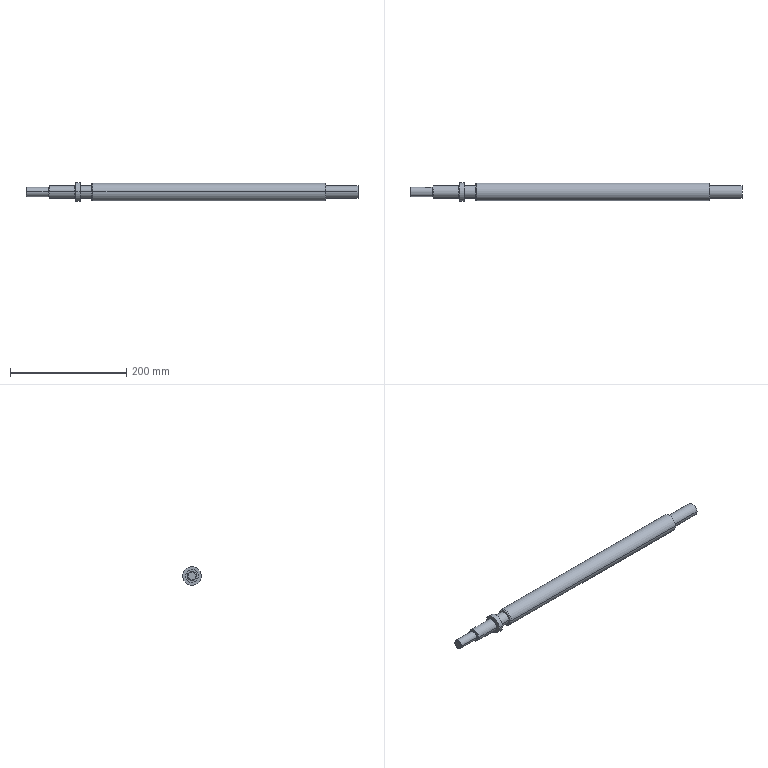Component | SolidWorks | 3LeadScrew-1 | 1 solid | 37 faces | box 570 x 32 x 32 mm | volume 343727 mm3 | cylinder 19 | plane 12 | cone 6 | commonest cylinder face diameters 22 x6 5 x3 16 x2 15 x2 21 x2 32 x2 30 x2
STEP:
#1=COLOUR_RGB('',0.7922,0.8196,0.9333);
#2=FILL_AREA_STYLE_COLOUR('',#1);
#3=FILL_AREA_STYLE('',(#2));
#4=SURFACE_STYLE_FILL_AREA(#3);
#5=SURFACE_SIDE_STYLE('',(#4));
#6=SURFACE_STYLE_USAGE(.BOTH.,#5);
#7=PRESENTATION_STYLE_ASSIGNMENT((#6));
#8=CARTESIAN_POINT('',(-12.116,2.748,-0.005406));
#9=VERTEX_POINT('',#8);
#10=CARTESIAN_POINT('',(-12.214,2.745,-0.1038));
#11=VERTEX_POINT('',#10);
#12=CARTESIAN_POINT('',(-12.214,2.748,-0.005406));
#13=DIRECTION('',(-0.,0.9996,-0.02861));
#14=DIRECTION('',(1.,0.,0.));
#15=AXIS2_PLACEMENT_3D('',#12,#13,#14);
#16=CIRCLE('',#15,0.09843);
#17=EDGE_CURVE('',#9,#11,#16,.T.);
#18=ORIENTED_EDGE('',*,*,#17,.F.);
#19=CARTESIAN_POINT('',(-12.116,2.874,-0.00901));
#20=VERTEX_POINT('',#19);
#21=CARTESIAN_POINT('',(-12.116,2.748,-0.005406));
#22=DIRECTION('',(-0.,0.9996,-0.02861));
#23=VECTOR('',#22,39.37);
#24=LINE('',#21,#23);
#25=EDGE_CURVE('',#9,#20,#24,.T.);
#26=ORIENTED_EDGE('',*,*,#25,.T.);
#27=CARTESIAN_POINT('',(-12.214,2.855,-0.1069));
#28=VERTEX_POINT('',#27);
#29=CARTESIAN_POINT('',(-12.214,2.855,-0.1069));
#30=CARTESIAN_POINT('',(-12.208,2.855,-0.1069));
#31=CARTESIAN_POINT('',(-12.201,2.856,-0.1063));
#32=CARTESIAN_POINT('',(-12.189,2.856,-0.1038));
#33=CARTESIAN_POINT('',(-12.182,2.857,-0.1019));
#34=CARTESIAN_POINT('',(-12.171,2.859,-0.09699));
#35=CARTESIAN_POINT('',(-12.165,2.86,-0.09399));
#36=CARTESIAN_POINT('',(-12.154,2.862,-0.0869));
#37=CARTESIAN_POINT('',(-12.149,2.863,-0.08281));
#38=CARTESIAN_POINT('',(-12.136,2.866,-0.06937));
#39=CARTESIAN_POINT('',(-12.128,2.869,-0.05851));
#40=CARTESIAN_POINT('',(-12.121,2.871,-0.04082));
#41=CARTESIAN_POINT('',(-12.119,2.872,-0.03459));
#42=CARTESIAN_POINT('',(-12.117,2.873,-0.02189));
#43=CARTESIAN_POINT('',(-12.116,2.874,-0.01548));
#44=CARTESIAN_POINT('',(-12.116,2.874,-0.00901));
#45=B_SPLINE_CURVE_WITH_KNOTS('',3,(#29,#30,#31,#32,#33,#34,#35,#36,#37,#38,#39,#40,#41,#42,#43,#44),.UNSPECIFIED.,.F.,.F.,(4,2,2,2,2,2,2,4),(0.,0.0004917,0.0009835,0.001475,0.001967,0.00295,0.003442,0.003934),.UNSPECIFIED.);
#46=EDGE_CURVE('',#28,#20,#45,.T.);
#47=ORIENTED_EDGE('',*,*,#46,.F.);
#48=CARTESIAN_POINT('',(-12.214,2.745,-0.1038));
#49=DIRECTION('',(-0.,0.9996,-0.02861));
#50=VECTOR('',#49,39.37);
#51=LINE('',#48,#50);
#52=EDGE_CURVE('',#11,#28,#51,.T.);
#53=ORIENTED_EDGE('',*,*,#52,.F.);
#54=EDGE_LOOP('',(#18,#26,#47,#53));
#55=FACE_OUTER_BOUND('',#54,.T.);
#56=CARTESIAN_POINT('',(-12.214,2.748,-0.005406));
#57=DIRECTION('',(-0.,0.9996,-0.02861));
#58=DIRECTION('',(1.,0.,0.));
#59=AXIS2_PLACEMENT_3D('',#56,#57,#58);
#60=CYLINDRICAL_SURFACE('',#59,0.09843);
#61=ADVANCED_FACE('',(#55),#60,.F.);
#62=CARTESIAN_POINT('',(-13.583,2.287,0.007791));
#63=VERTEX_POINT('',#62);
#64=CARTESIAN_POINT('',(-13.583,2.831,-0.007791));
#65=VERTEX_POINT('',#64);
#66=CARTESIAN_POINT('',(-13.583,2.559,-0.));
#67=DIRECTION('',(1.,0.,0.));
#68=DIRECTION('',(0.,-0.9996,0.02861));
#69=AXIS2_PLACEMENT_3D('',#66,#67,#68);
#70=CIRCLE('',#69,0.2723);
#71=EDGE_CURVE('',#63,#65,#70,.T.);
#72=ORIENTED_EDGE('',*,*,#71,.T.);
#73=CARTESIAN_POINT('',(-13.54,2.874,-0.00901));
#74=VERTEX_POINT('',#73);
#75=CARTESIAN_POINT('',(-13.583,2.831,-0.007791));
#76=DIRECTION('',(0.7071,0.7068,-0.02023));
#77=VECTOR('',#76,39.37);
#78=LINE('',#75,#77);
#79=EDGE_CURVE('',#65,#74,#78,.T.);
#80=ORIENTED_EDGE('',*,*,#79,.T.);
#81=CARTESIAN_POINT('',(-13.54,2.244,0.00901));
#82=VERTEX_POINT('',#81);
#83=CARTESIAN_POINT('',(-13.54,2.559,-0.));
#84=DIRECTION('',(1.,0.,0.));
#85=DIRECTION('',(0.,-0.9996,0.02861));
#86=AXIS2_PLACEMENT_3D('',#83,#84,#85);
#87=CIRCLE('',#86,0.315);
#88=EDGE_CURVE('',#82,#74,#87,.T.);
#89=ORIENTED_EDGE('',*,*,#88,.F.);
#90=CARTESIAN_POINT('',(-13.583,2.287,0.007791));
#91=DIRECTION('',(0.7071,-0.7068,0.02023));
#92=VECTOR('',#91,39.37);
#93=LINE('',#90,#92);
#94=EDGE_CURVE('',#63,#82,#93,.T.);
#95=ORIENTED_EDGE('',*,*,#94,.F.);
#96=EDGE_LOOP('',(#72,#80,#89,#95));
#97=FACE_OUTER_BOUND('',#96,.T.);
#98=CARTESIAN_POINT('',(-13.583,2.559,-0.));
#99=DIRECTION('',(1.,0.,0.));
#100=DIRECTION('',(0.,-0.9996,0.02861));
#101=AXIS2_PLACEMENT_3D('',#98,#99,#100);
#102=CONICAL_SURFACE('',#101,0.2723,0.7854);
#103=ADVANCED_FACE('',(#97),#102,.T.);
#104=CARTESIAN_POINT('',(-9.134,3.104,-0.01559));
#105=VERTEX_POINT('',#104);
#106=CARTESIAN_POINT('',(-9.134,2.014,0.01559));
#107=VERTEX_POINT('',#106);
#108=CARTESIAN_POINT('',(-9.134,2.559,-0.));
#109=DIRECTION('',(-1.,-0.,-0.));
#110=DIRECTION('',(0.,0.9996,-0.02861));
#111=AXIS2_PLACEMENT_3D('',#108,#109,#110);
#112=CIRCLE('',#111,0.5451);
#113=EDGE_CURVE('',#105,#107,#112,.T.);
#114=ORIENTED_EDGE('',*,*,#113,.F.);
#115=CARTESIAN_POINT('',(-9.055,3.149,-0.01689));
#116=VERTEX_POINT('',#115);
#117=CARTESIAN_POINT('',(-9.134,3.104,-0.01559));
#118=DIRECTION('',(0.866,0.4998,-0.0143));
#119=VECTOR('',#118,39.37);
#120=LINE('',#117,#119);
#121=EDGE_CURVE('',#105,#116,#120,.T.);
#122=ORIENTED_EDGE('',*,*,#121,.T.);
#123=CARTESIAN_POINT('',(-9.055,1.969,0.01689));
#124=VERTEX_POINT('',#123);
#125=CARTESIAN_POINT('',(-9.055,2.559,-0.));
#126=DIRECTION('',(1.,0.,0.));
#127=DIRECTION('',(0.,0.9996,-0.02861));
#128=AXIS2_PLACEMENT_3D('',#125,#126,#127);
#129=CIRCLE('',#128,0.5906);
#130=EDGE_CURVE('',#124,#116,#129,.T.);
#131=ORIENTED_EDGE('',*,*,#130,.F.);
#132=CARTESIAN_POINT('',(-9.134,2.014,0.01559));
#133=DIRECTION('',(0.866,-0.4998,0.0143));
#134=VECTOR('',#133,39.37);
#135=LINE('',#132,#134);
#136=EDGE_CURVE('',#107,#124,#135,.T.);
#137=ORIENTED_EDGE('',*,*,#136,.F.);
#138=EDGE_LOOP('',(#114,#122,#131,#137));
#139=FACE_OUTER_BOUND('',#138,.T.);
#140=CARTESIAN_POINT('',(-9.134,2.559,-0.));
#141=DIRECTION('',(1.,0.,0.));
#142=DIRECTION('',(0.,-0.9996,0.02861));
#143=AXIS2_PLACEMENT_3D('',#140,#141,#142);
#144=CONICAL_SURFACE('',#143,0.5451,0.5236);
#145=ADVANCED_FACE('',(#139),#144,.T.);
#146=CARTESIAN_POINT('',(6.693,2.047,0.01464));
#147=VERTEX_POINT('',#146);
#148=CARTESIAN_POINT('',(6.693,3.071,-0.01464));
#149=VERTEX_POINT('',#148);
#150=CARTESIAN_POINT('',(6.693,2.559,-0.));
#151=DIRECTION('',(1.,0.,0.));
#152=DIRECTION('',(0.,0.9996,-0.02861));
#153=AXIS2_PLACEMENT_3D('',#150,#151,#152);
#154=CIRCLE('',#153,0.5118);
#155=EDGE_CURVE('',#147,#149,#154,.T.);
#156=ORIENTED_EDGE('',*,*,#155,.F.);
#157=CARTESIAN_POINT('',(6.647,1.969,0.01689));
#158=VERTEX_POINT('',#157);
#159=CARTESIAN_POINT('',(6.647,1.969,0.01689));
#160=DIRECTION('',(-0.5,-0.8657,0.02477));
#161=VECTOR('',#160,39.37);
#162=LINE('',#159,#161);
#163=EDGE_CURVE('',#147,#158,#162,.T.);
#164=ORIENTED_EDGE('',*,*,#163,.T.);
#165=CARTESIAN_POINT('',(6.647,3.149,-0.01689));
#166=VERTEX_POINT('',#165);
#167=CARTESIAN_POINT('',(6.647,2.559,-0.));
#168=DIRECTION('',(-1.,-0.,-0.));
#169=DIRECTION('',(0.,0.9996,-0.02861));
#170=AXIS2_PLACEMENT_3D('',#167,#168,#169);
#171=CIRCLE('',#170,0.5906);
#172=EDGE_CURVE('',#166,#158,#171,.T.);
#173=ORIENTED_EDGE('',*,*,#172,.F.);
#174=CARTESIAN_POINT('',(6.647,3.149,-0.01689));
#175=DIRECTION('',(-0.5,0.8657,-0.02477));
#176=VECTOR('',#175,39.37);
#177=LINE('',#174,#176);
#178=EDGE_CURVE('',#149,#166,#177,.T.);
#179=ORIENTED_EDGE('',*,*,#178,.F.);
#180=EDGE_LOOP('',(#156,#164,#173,#179));
#181=FACE_OUTER_BOUND('',#180,.T.);
#182=CARTESIAN_POINT('',(6.647,2.559,-0.));
#183=DIRECTION('',(-1.,-0.,-0.));
#184=DIRECTION('',(0.,0.9996,-0.02861));
#185=AXIS2_PLACEMENT_3D('',#182,#183,#184);
#186=CONICAL_SURFACE('',#185,0.5906,1.047);
#187=ADVANCED_FACE('',(#181),#186,.T.);
#188=ORIENTED_EDGE('',*,*,#88,.T.);
#189=CARTESIAN_POINT('',(-12.588,2.874,-0.00901));
#190=VERTEX_POINT('',#189);
#191=CARTESIAN_POINT('',(-13.583,2.874,-0.00901));
#192=DIRECTION('',(1.,0.,0.));
#193=VECTOR('',#192,39.37);
#194=LINE('',#191,#193);
#195=EDGE_CURVE('',#74,#190,#194,.T.);
#196=ORIENTED_EDGE('',*,*,#195,.T.);
#197=CARTESIAN_POINT('',(-12.49,2.855,-0.1069));
#198=VERTEX_POINT('',#197);
#199=CARTESIAN_POINT('',(-12.588,2.874,-0.00901));
#200=CARTESIAN_POINT('',(-12.588,2.874,-0.01547));
#201=CARTESIAN_POINT('',(-12.588,2.873,-0.02202));
#202=CARTESIAN_POINT('',(-12.585,2.872,-0.03464));
#203=CARTESIAN_POINT('',(-12.583,2.871,-0.04077));
#204=CARTESIAN_POINT('',(-12.578,2.87,-0.05269));
#205=CARTESIAN_POINT('',(-12.575,2.869,-0.05835));
#206=CARTESIAN_POINT('',(-12.568,2.866,-0.0689));
#207=CARTESIAN_POINT('',(-12.564,2.865,-0.07387));
#208=CARTESIAN_POINT('',(-12.555,2.863,-0.08287));
#209=CARTESIAN_POINT('',(-12.55,2.862,-0.08688));
#210=CARTESIAN_POINT('',(-12.539,2.86,-0.09395));
#211=CARTESIAN_POINT('',(-12.534,2.859,-0.09701));
#212=CARTESIAN_POINT('',(-12.522,2.857,-0.1019));
#213=CARTESIAN_POINT('',(-12.516,2.856,-0.1038));
#214=CARTESIAN_POINT('',(-12.503,2.856,-0.1063));
#215=CARTESIAN_POINT('',(-12.496,2.855,-0.1069));
#216=CARTESIAN_POINT('',(-12.49,2.855,-0.1069));
#217=B_SPLINE_CURVE_WITH_KNOTS('',3,(#199,#200,#201,#202,#203,#204,#205,#206,#207,#208,#209,#210,#211,#212,#213,#214,#215,#216),.UNSPECIFIED.,.F.,.F.,(4,2,2,2,2,2,2,2,4),(0.003934,0.004425,0.004916,0.005407,0.005898,0.006389,0.006881,0.007372,0.007863),.UNSPECIFIED.);
#218=EDGE_CURVE('',#190,#198,#217,.T.);
#219=ORIENTED_EDGE('',*,*,#218,.T.);
#220=CARTESIAN_POINT('',(-13.583,2.855,-0.1069));
#221=DIRECTION('',(1.,0.,0.));
#222=VECTOR('',#221,39.37);
#223=LINE('',#220,#222);
#224=EDGE_CURVE('',#198,#28,#223,.T.);
#225=ORIENTED_EDGE('',*,*,#224,.T.);
#226=ORIENTED_EDGE('',*,*,#46,.T.);
#227=CARTESIAN_POINT('',(-12.087,2.874,-0.00901));
#228=VERTEX_POINT('',#227);
#229=CARTESIAN_POINT('',(-13.583,2.874,-0.00901));
#230=DIRECTION('',(1.,0.,0.));
#231=VECTOR('',#230,39.37);
#232=LINE('',#229,#231);
#233=EDGE_CURVE('',#20,#228,#232,.T.);
#234=ORIENTED_EDGE('',*,*,#233,.T.);
#235=CARTESIAN_POINT('',(-12.087,2.244,0.00901));
#236=VERTEX_POINT('',#235);
#237=CARTESIAN_POINT('',(-12.087,2.559,-0.));
#238=DIRECTION('',(-1.,-0.,-0.));
#239=DIRECTION('',(0.,0.9996,-0.02861));
#240=AXIS2_PLACEMENT_3D('',#237,#238,#239);
#241=CIRCLE('',#240,0.315);
#242=EDGE_CURVE('',#228,#236,#241,.T.);
#243=ORIENTED_EDGE('',*,*,#242,.T.);
#244=CARTESIAN_POINT('',(-13.583,2.244,0.00901));
#245=DIRECTION('',(1.,0.,0.));
#246=VECTOR('',#245,39.37);
#247=LINE('',#244,#246);
#248=EDGE_CURVE('',#82,#236,#247,.T.);
#249=ORIENTED_EDGE('',*,*,#248,.F.);
#250=EDGE_LOOP('',(#188,#196,#219,#225,#226,#234,#243,#249));
#251=FACE_OUTER_BOUND('',#250,.T.);
#252=CARTESIAN_POINT('',(-13.583,2.559,-0.));
#253=DIRECTION('',(1.,0.,0.));
#254=DIRECTION('',(0.,-0.9996,0.02861));
#255=AXIS2_PLACEMENT_3D('',#252,#253,#254);
#256=CYLINDRICAL_SURFACE('',#255,0.315);
#257=ADVANCED_FACE('',(#251),#256,.T.);
#258=CARTESIAN_POINT('',(-12.087,2.854,-0.008447));
#259=VERTEX_POINT('',#258);
#260=CARTESIAN_POINT('',(-12.087,2.264,0.008447));
#261=VERTEX_POINT('',#260);
#262=CARTESIAN_POINT('',(-12.087,2.559,-0.));
#263=DIRECTION('',(-1.,-0.,-0.));
#264=DIRECTION('',(0.,0.9996,-0.02861));
#265=AXIS2_PLACEMENT_3D('',#262,#263,#264);
#266=CIRCLE('',#265,0.2953);
#267=EDGE_CURVE('',#259,#261,#266,.T.);
#268=ORIENTED_EDGE('',*,*,#267,.F.);
#269=CARTESIAN_POINT('',(-12.008,2.854,-0.008447));
#270=VERTEX_POINT('',#269);
#271=CARTESIAN_POINT('',(-12.087,2.854,-0.008447));
#272=DIRECTION('',(1.,0.,0.));
#273=VECTOR('',#272,39.37);
#274=LINE('',#271,#273);
#275=EDGE_CURVE('',#259,#270,#274,.T.);
#276=ORIENTED_EDGE('',*,*,#275,.T.);
#277=CARTESIAN_POINT('',(-12.008,2.264,0.008447));
#278=VERTEX_POINT('',#277);
#279=CARTESIAN_POINT('',(-12.008,2.559,-0.));
#280=DIRECTION('',(-1.,-0.,-0.));
#281=DIRECTION('',(0.,0.9996,-0.02861));
#282=AXIS2_PLACEMENT_3D('',#279,#280,#281);
#283=CIRCLE('',#282,0.2953);
#284=EDGE_CURVE('',#270,#278,#283,.T.);
#285=ORIENTED_EDGE('',*,*,#284,.T.);
#286=CARTESIAN_POINT('',(-12.087,2.264,0.008447));
#287=DIRECTION('',(1.,0.,0.));
#288=VECTOR('',#287,39.37);
#289=LINE('',#286,#288);
#290=EDGE_CURVE('',#261,#278,#289,.T.);
#291=ORIENTED_EDGE('',*,*,#290,.F.);
#292=EDGE_LOOP('',(#268,#276,#285,#291));
#293=FACE_OUTER_BOUND('',#292,.T.);
#294=CARTESIAN_POINT('',(-12.087,2.559,-0.));
#295=DIRECTION('',(1.,0.,0.));
#296=DIRECTION('',(0.,-0.9996,0.02861));
#297=AXIS2_PLACEMENT_3D('',#294,#295,#296);
#298=CYLINDRICAL_SURFACE('',#297,0.2953);
#299=ADVANCED_FACE('',(#293),#298,.T.);
#300=CARTESIAN_POINT('',(-12.008,2.992,-0.01239));
#301=VERTEX_POINT('',#300);
#302=CARTESIAN_POINT('',(-12.008,2.126,0.01239));
#303=VERTEX_POINT('',#302);
#304=CARTESIAN_POINT('',(-12.008,2.559,-0.));
#305=DIRECTION('',(-1.,-0.,-0.));
#306=DIRECTION('',(0.,0.9996,-0.02861));
#307=AXIS2_PLACEMENT_3D('',#304,#305,#306);
#308=CIRCLE('',#307,0.4331);
#309=EDGE_CURVE('',#301,#303,#308,.T.);
#310=ORIENTED_EDGE('',*,*,#309,.F.);
#311=CARTESIAN_POINT('',(-10.315,2.992,-0.01239));
#312=VERTEX_POINT('',#311);
#313=CARTESIAN_POINT('',(-12.008,2.992,-0.01239));
#314=DIRECTION('',(1.,0.,0.));
#315=VECTOR('',#314,39.37);
#316=LINE('',#313,#315);
#317=EDGE_CURVE('',#301,#312,#316,.T.);
#318=ORIENTED_EDGE('',*,*,#317,.T.);
#319=CARTESIAN_POINT('',(-10.315,2.126,0.01239));
#320=VERTEX_POINT('',#319);
#321=CARTESIAN_POINT('',(-10.315,2.559,-0.));
#322=DIRECTION('',(-1.,-0.,-0.));
#323=DIRECTION('',(0.,0.9996,-0.02861));
#324=AXIS2_PLACEMENT_3D('',#321,#322,#323);
#325=CIRCLE('',#324,0.4331);
#326=EDGE_CURVE('',#312,#320,#325,.T.);
#327=ORIENTED_EDGE('',*,*,#326,.T.);
#328=CARTESIAN_POINT('',(-12.008,2.126,0.01239));
#329=DIRECTION('',(1.,0.,0.));
#330=VECTOR('',#329,39.37);
#331=LINE('',#328,#330);
#332=EDGE_CURVE('',#303,#320,#331,.T.);
#333=ORIENTED_EDGE('',*,*,#332,.F.);
#334=EDGE_LOOP('',(#310,#318,#327,#333));
#335=FACE_OUTER_BOUND('',#334,.T.);
#336=CARTESIAN_POINT('',(-12.008,2.559,-0.));
#337=DIRECTION('',(1.,0.,0.));
#338=DIRECTION('',(0.,-0.9996,0.02861));
#339=AXIS2_PLACEMENT_3D('',#336,#337,#338);
#340=CYLINDRICAL_SURFACE('',#339,0.4331);
#341=ADVANCED_FACE('',(#335),#340,.T.);
#342=CARTESIAN_POINT('',(-10.315,2.972,-0.01183));
#343=VERTEX_POINT('',#342);
#344=CARTESIAN_POINT('',(-10.315,2.146,0.01183));
#345=VERTEX_POINT('',#344);
#346=CARTESIAN_POINT('',(-10.315,2.559,-0.));
#347=DIRECTION('',(-1.,-0.,-0.));
#348=DIRECTION('',(0.,0.9996,-0.02861));
#349=AXIS2_PLACEMENT_3D('',#346,#347,#348);
#350=CIRCLE('',#349,0.4134);
#351=EDGE_CURVE('',#343,#345,#350,.T.);
#352=ORIENTED_EDGE('',*,*,#351,.F.);
#353=CARTESIAN_POINT('',(-10.236,2.972,-0.01183));
#354=VERTEX_POINT('',#353);
#355=CARTESIAN_POINT('',(-10.315,2.972,-0.01183));
#356=DIRECTION('',(1.,0.,0.));
#357=VECTOR('',#356,39.37);
#358=LINE('',#355,#357);
#359=EDGE_CURVE('',#343,#354,#358,.T.);
#360=ORIENTED_EDGE('',*,*,#359,.T.);
#361=CARTESIAN_POINT('',(-10.236,2.146,0.01183));
#362=VERTEX_POINT('',#361);
#363=CARTESIAN_POINT('',(-10.236,2.559,-0.));
#364=DIRECTION('',(-1.,-0.,-0.));
#365=DIRECTION('',(0.,0.9996,-0.02861));
#366=AXIS2_PLACEMENT_3D('',#363,#364,#365);
#367=CIRCLE('',#366,0.4134);
#368=EDGE_CURVE('',#354,#362,#367,.T.);
#369=ORIENTED_EDGE('',*,*,#368,.T.);
#370=CARTESIAN_POINT('',(-10.315,2.146,0.01183));
#371=DIRECTION('',(1.,0.,0.));
#372=VECTOR('',#371,39.37);
#373=LINE('',#370,#372);
#374=EDGE_CURVE('',#345,#362,#373,.T.);
#375=ORIENTED_EDGE('',*,*,#374,.F.);
#376=EDGE_LOOP('',(#352,#360,#369,#375));
#377=FACE_OUTER_BOUND('',#376,.T.);
#378=CARTESIAN_POINT('',(-10.315,2.559,-0.));
#379=DIRECTION('',(1.,0.,0.));
#380=DIRECTION('',(0.,-0.9996,0.02861));
#381=AXIS2_PLACEMENT_3D('',#378,#379,#380);
#382=CYLINDRICAL_SURFACE('',#381,0.4134);
#383=ADVANCED_FACE('',(#377),#382,.T.);
#384=CARTESIAN_POINT('',(-10.236,3.189,-0.01802));
#385=VERTEX_POINT('',#384);
#386=CARTESIAN_POINT('',(-10.236,1.929,0.01802));
#387=VERTEX_POINT('',#386);
#388=CARTESIAN_POINT('',(-10.236,2.559,-0.));
#389=DIRECTION('',(-1.,-0.,-0.));
#390=DIRECTION('',(0.,0.9996,-0.02861));
#391=AXIS2_PLACEMENT_3D('',#388,#389,#390);
#392=CIRCLE('',#391,0.6299);
#393=EDGE_CURVE('',#385,#387,#392,.T.);
#394=ORIENTED_EDGE('',*,*,#393,.F.);
#395=CARTESIAN_POINT('',(-9.921,3.189,-0.01802));
#396=VERTEX_POINT('',#395);
#397=CARTESIAN_POINT('',(-10.236,3.189,-0.01802));
#398=DIRECTION('',(1.,0.,0.));
#399=VECTOR('',#398,39.37);
#400=LINE('',#397,#399);
#401=EDGE_CURVE('',#385,#396,#400,.T.);
#402=ORIENTED_EDGE('',*,*,#401,.T.);
#403=CARTESIAN_POINT('',(-9.921,1.929,0.01802));
#404=VERTEX_POINT('',#403);
#405=CARTESIAN_POINT('',(-9.921,2.559,-0.));
#406=DIRECTION('',(-1.,-0.,-0.));
#407=DIRECTION('',(0.,0.9996,-0.02861));
#408=AXIS2_PLACEMENT_3D('',#405,#406,#407);
#409=CIRCLE('',#408,0.6299);
#410=EDGE_CURVE('',#396,#404,#409,.T.);
#411=ORIENTED_EDGE('',*,*,#410,.T.);
#412=CARTESIAN_POINT('',(-10.236,1.929,0.01802));
#413=DIRECTION('',(1.,0.,0.));
#414=VECTOR('',#413,39.37);
#415=LINE('',#412,#414);
#416=EDGE_CURVE('',#387,#404,#415,.T.);
#417=ORIENTED_EDGE('',*,*,#416,.F.);
#418=EDGE_LOOP('',(#394,#402,#411,#417));
#419=FACE_OUTER_BOUND('',#418,.T.);
#420=CARTESIAN_POINT('',(-10.236,2.559,-0.));
#421=DIRECTION('',(1.,0.,0.));
#422=DIRECTION('',(0.,-0.9996,0.02861));
#423=AXIS2_PLACEMENT_3D('',#420,#421,#422);
#424=CYLINDRICAL_SURFACE('',#423,0.6299);
#425=ADVANCED_FACE('',(#419),#424,.T.);
#426=CARTESIAN_POINT('',(-9.921,2.992,-0.01239));
#427=VERTEX_POINT('',#426);
#428=CARTESIAN_POINT('',(-9.921,2.126,0.01239));
#429=VERTEX_POINT('',#428);
#430=CARTESIAN_POINT('',(-9.921,2.559,-0.));
#431=DIRECTION('',(-1.,-0.,-0.));
#432=DIRECTION('',(0.,0.9996,-0.02861));
#433=AXIS2_PLACEMENT_3D('',#430,#431,#432);
#434=CIRCLE('',#433,0.4331);
#435=EDGE_CURVE('',#427,#429,#434,.T.);
#436=ORIENTED_EDGE('',*,*,#435,.F.);
#437=CARTESIAN_POINT('',(-9.134,2.992,-0.01239));
#438=VERTEX_POINT('',#437);
#439=CARTESIAN_POINT('',(-9.921,2.992,-0.01239));
#440=DIRECTION('',(1.,0.,0.));
#441=VECTOR('',#440,39.37);
#442=LINE('',#439,#441);
#443=EDGE_CURVE('',#427,#438,#442,.T.);
#444=ORIENTED_EDGE('',*,*,#443,.T.);
#445=CARTESIAN_POINT('',(-9.134,2.126,0.01239));
#446=VERTEX_POINT('',#445);
#447=CARTESIAN_POINT('',(-9.134,2.559,-0.));
#448=DIRECTION('',(-1.,-0.,-0.));
#449=DIRECTION('',(0.,0.9996,-0.02861));
#450=AXIS2_PLACEMENT_3D('',#447,#448,#449);
#451=CIRCLE('',#450,0.4331);
#452=EDGE_CURVE('',#438,#446,#451,.T.);
#453=ORIENTED_EDGE('',*,*,#452,.T.);
#454=CARTESIAN_POINT('',(-9.921,2.126,0.01239));
#455=DIRECTION('',(1.,0.,0.));
#456=VECTOR('',#455,39.37);
#457=LINE('',#454,#456);
#458=EDGE_CURVE('',#429,#446,#457,.T.);
#459=ORIENTED_EDGE('',*,*,#458,.F.);
#460=EDGE_LOOP('',(#436,#444,#453,#459));
#461=FACE_OUTER_BOUND('',#460,.T.);
#462=CARTESIAN_POINT('',(-9.921,2.559,-0.));
#463=DIRECTION('',(1.,0.,0.));
#464=DIRECTION('',(0.,-0.9996,0.02861));
#465=AXIS2_PLACEMENT_3D('',#462,#463,#464);
#466=CYLINDRICAL_SURFACE('',#465,0.4331);
#467=ADVANCED_FACE('',(#461),#466,.T.);
#468=ORIENTED_EDGE('',*,*,#130,.T.);
#469=CARTESIAN_POINT('',(-9.134,3.149,-0.01689));
#470=DIRECTION('',(1.,0.,0.));
#471=VECTOR('',#470,39.37);
#472=LINE('',#469,#471);
#473=EDGE_CURVE('',#116,#166,#472,.T.);
#474=ORIENTED_EDGE('',*,*,#473,.T.);
#475=ORIENTED_EDGE('',*,*,#172,.T.);
#476=CARTESIAN_POINT('',(-9.134,1.969,0.01689));
#477=DIRECTION('',(1.,0.,0.));
#478=VECTOR('',#477,39.37);
#479=LINE('',#476,#478);
#480=EDGE_CURVE('',#124,#158,#479,.T.);
#481=ORIENTED_EDGE('',*,*,#480,.F.);
#482=EDGE_LOOP('',(#468,#474,#475,#481));
#483=FACE_OUTER_BOUND('',#482,.T.);
#484=CARTESIAN_POINT('',(-9.134,2.559,-0.));
#485=DIRECTION('',(1.,0.,0.));
#486=DIRECTION('',(0.,-0.9996,0.02861));
#487=AXIS2_PLACEMENT_3D('',#484,#485,#486);
#488=CYLINDRICAL_SURFACE('',#487,0.5906);
#489=ADVANCED_FACE('',(#483),#488,.T.);
#490=CARTESIAN_POINT('',(6.693,2.992,-0.01239));
#491=VERTEX_POINT('',#490);
#492=CARTESIAN_POINT('',(6.693,2.126,0.01239));
#493=VERTEX_POINT('',#492);
#494=CARTESIAN_POINT('',(6.693,2.559,-0.));
#495=DIRECTION('',(-1.,-0.,-0.));
#496=DIRECTION('',(0.,0.9996,-0.02861));
#497=AXIS2_PLACEMENT_3D('',#494,#495,#496);
#498=CIRCLE('',#497,0.4331);
#499=EDGE_CURVE('',#491,#493,#498,.T.);
#500=ORIENTED_EDGE('',*,*,#499,.F.);
#501=CARTESIAN_POINT('',(8.858,2.992,-0.01239));
#502=VERTEX_POINT('',#501);
#503=CARTESIAN_POINT('',(6.693,2.992,-0.01239));
#504=DIRECTION('',(1.,0.,0.));
#505=VECTOR('',#504,39.37);
#506=LINE('',#503,#505);
#507=EDGE_CURVE('',#491,#502,#506,.T.);
#508=ORIENTED_EDGE('',*,*,#507,.T.);
#509=CARTESIAN_POINT('',(8.858,2.126,0.01239));
#510=VERTEX_POINT('',#509);
#511=CARTESIAN_POINT('',(8.858,2.559,-0.));
#512=DIRECTION('',(-1.,-0.,-0.));
#513=DIRECTION('',(0.,0.9996,-0.02861));
#514=AXIS2_PLACEMENT_3D('',#511,#512,#513);
#515=CIRCLE('',#514,0.4331);
#516=EDGE_CURVE('',#502,#510,#515,.T.);
#517=ORIENTED_EDGE('',*,*,#516,.T.);
#518=CARTESIAN_POINT('',(6.693,2.126,0.01239));
#519=DIRECTION('',(1.,0.,0.));
#520=VECTOR('',#519,39.37);
#521=LINE('',#518,#520);
#522=EDGE_CURVE('',#493,#510,#521,.T.);
#523=ORIENTED_EDGE('',*,*,#522,.F.);
#524=EDGE_LOOP('',(#500,#508,#517,#523));
#525=FACE_OUTER_BOUND('',#524,.T.);
#526=CARTESIAN_POINT('',(6.693,2.559,-0.));
#527=DIRECTION('',(1.,0.,0.));
#528=DIRECTION('',(0.,-0.9996,0.02861));
#529=AXIS2_PLACEMENT_3D('',#526,#527,#528);
#530=CYLINDRICAL_SURFACE('',#529,0.4331);
#531=ADVANCED_FACE('',(#525),#530,.T.);
#532=ORIENTED_EDGE('',*,*,#507,.F.);
#533=CARTESIAN_POINT('',(6.693,2.559,-0.));
#534=DIRECTION('',(-1.,-0.,-0.));
#535=DIRECTION('',(0.,0.9996,-0.02861));
#536=AXIS2_PLACEMENT_3D('',#533,#534,#535);
#537=CIRCLE('',#536,0.4331);
#538=EDGE_CURVE('',#493,#491,#537,.T.);
#539=ORIENTED_EDGE('',*,*,#538,.F.);
#540=ORIENTED_EDGE('',*,*,#522,.T.);
#541=CARTESIAN_POINT('',(8.858,2.559,-0.));
#542=DIRECTION('',(-1.,-0.,-0.));
#543=DIRECTION('',(0.,0.9996,-0.02861));
#544=AXIS2_PLACEMENT_3D('',#541,#542,#543);
#545=CIRCLE('',#544,0.4331);
#546=EDGE_CURVE('',#510,#502,#545,.T.);
#547=ORIENTED_EDGE('',*,*,#546,.T.);
#548=EDGE_LOOP('',(#532,#539,#540,#547));
#549=FACE_OUTER_BOUND('',#548,.T.);
#550=CARTESIAN_POINT('',(6.693,2.559,-0.));
#551=DIRECTION('',(1.,0.,0.));
#552=DIRECTION('',(0.,-0.9996,0.02861));
#553=AXIS2_PLACEMENT_3D('',#550,#551,#552);
#554=CYLINDRICAL_SURFACE('',#553,0.4331);
#555=ADVANCED_FACE('',(#549),#554,.T.);
#556=ORIENTED_EDGE('',*,*,#546,.F.);
#557=ORIENTED_EDGE('',*,*,#516,.F.);
#558=EDGE_LOOP('',(#556,#557));
#559=FACE_OUTER_BOUND('',#558,.T.);
#560=CARTESIAN_POINT('',(8.858,2.559,-0.));
#561=DIRECTION('',(-1.,-0.,-0.));
#562=DIRECTION('',(-0.,0.9996,-0.02861));
#563=AXIS2_PLACEMENT_3D('',#560,#561,#562);
#564=PLANE('',#563);
#565=ADVANCED_FACE('',(#559),#564,.F.);
#566=ORIENTED_EDGE('',*,*,#473,.F.);
#567=CARTESIAN_POINT('',(-9.055,2.559,-0.));
#568=DIRECTION('',(1.,0.,0.));
#569=DIRECTION('',(0.,0.9996,-0.02861));
#570=AXIS2_PLACEMENT_3D('',#567,#568,#569);
#571=CIRCLE('',#570,0.5906);
#572=EDGE_CURVE('',#116,#124,#571,.T.);
#573=ORIENTED_EDGE('',*,*,#572,.T.);
#574=ORIENTED_EDGE('',*,*,#480,.T.);
#575=CARTESIAN_POINT('',(6.647,2.559,-0.));
#576=DIRECTION('',(-1.,-0.,-0.));
#577=DIRECTION('',(0.,0.9996,-0.02861));
#578=AXIS2_PLACEMENT_3D('',#575,#576,#577);
#579=CIRCLE('',#578,0.5906);
#580=EDGE_CURVE('',#158,#166,#579,.T.);
#581=ORIENTED_EDGE('',*,*,#580,.T.);
#582=EDGE_LOOP('',(#566,#573,#574,#581));
#583=FACE_OUTER_BOUND('',#582,.T.);
#584=CARTESIAN_POINT('',(-9.134,2.559,-0.));
#585=DIRECTION('',(1.,0.,0.));
#586=DIRECTION('',(0.,-0.9996,0.02861));
#587=AXIS2_PLACEMENT_3D('',#584,#585,#586);
#588=CYLINDRICAL_SURFACE('',#587,0.5906);
#589=ADVANCED_FACE('',(#583),#588,.T.);
#590=CARTESIAN_POINT('',(-9.134,2.559,-0.));
#591=DIRECTION('',(-1.,-0.,-0.));
#592=DIRECTION('',(0.,0.9996,-0.02861));
#593=AXIS2_PLACEMENT_3D('',#590,#591,#592);
#594=CIRCLE('',#593,0.5451);
#595=EDGE_CURVE('',#107,#105,#594,.T.);
#596=ORIENTED_EDGE('',*,*,#595,.T.);
#597=ORIENTED_EDGE('',*,*,#113,.T.);
#598=EDGE_LOOP('',(#596,#597));
#599=FACE_OUTER_BOUND('',#598,.T.);
#600=CARTESIAN_POINT('',(-9.134,2.559,-0.));
#601=DIRECTION('',(-1.,-0.,-0.));
#602=DIRECTION('',(0.,0.9996,-0.02861));
#603=AXIS2_PLACEMENT_3D('',#600,#601,#602);
#604=CIRCLE('',#603,0.4331);
#605=EDGE_CURVE('',#446,#438,#604,.T.);
#606=ORIENTED_EDGE('',*,*,#605,.F.);
#607=ORIENTED_EDGE('',*,*,#452,.F.);
#608=EDGE_LOOP('',(#606,#607));
#609=FACE_BOUND('',#608,.T.);
#610=CARTESIAN_POINT('',(-9.134,2.559,-0.));
#611=DIRECTION('',(-1.,-0.,-0.));
#612=DIRECTION('',(-0.,0.9996,-0.02861));
#613=AXIS2_PLACEMENT_3D('',#610,#611,#612);
#614=PLANE('',#613);
#615=ADVANCED_FACE('',(#599,#609),#614,.T.);
#616=CARTESIAN_POINT('',(6.693,2.559,-0.));
#617=DIRECTION('',(1.,0.,0.));
#618=DIRECTION('',(0.,0.9996,-0.02861));
#619=AXIS2_PLACEMENT_3D('',#616,#617,#618);
#620=CIRCLE('',#619,0.5118);
#621=EDGE_CURVE('',#149,#147,#620,.T.);
#622=ORIENTED_EDGE('',*,*,#621,.T.);
#623=ORIENTED_EDGE('',*,*,#155,.T.);
#624=EDGE_LOOP('',(#622,#623));
#625=FACE_OUTER_BOUND('',#624,.T.);
#626=ORIENTED_EDGE('',*,*,#538,.T.);
#627=ORIENTED_EDGE('',*,*,#499,.T.);
#628=EDGE_LOOP('',(#626,#627));
#629=FACE_BOUND('',#628,.T.);
#630=CARTESIAN_POINT('',(6.693,2.559,-0.));
#631=DIRECTION('',(-1.,-0.,-0.));
#632=DIRECTION('',(-0.,0.9996,-0.02861));
#633=AXIS2_PLACEMENT_3D('',#630,#631,#632);
#634=PLANE('',#633);
#635=ADVANCED_FACE('',(#625,#629),#634,.F.);
#636=ORIENTED_EDGE('',*,*,#443,.F.);
#637=CARTESIAN_POINT('',(-9.921,2.559,-0.));
#638=DIRECTION('',(-1.,-0.,-0.));
#639=DIRECTION('',(0.,0.9996,-0.02861));
#640=AXIS2_PLACEMENT_3D('',#637,#638,#639);
#641=CIRCLE('',#640,0.4331);
#642=EDGE_CURVE('',#429,#427,#641,.T.);
#643=ORIENTED_EDGE('',*,*,#642,.F.);
#644=ORIENTED_EDGE('',*,*,#458,.T.);
#645=ORIENTED_EDGE('',*,*,#605,.T.);
#646=EDGE_LOOP('',(#636,#643,#644,#645));
#647=FACE_OUTER_BOUND('',#646,.T.);
#648=CARTESIAN_POINT('',(-9.921,2.559,-0.));
#649=DIRECTION('',(1.,0.,0.));
#650=DIRECTION('',(0.,-0.9996,0.02861));
#651=AXIS2_PLACEMENT_3D('',#648,#649,#650);
#652=CYLINDRICAL_SURFACE('',#651,0.4331);
#653=ADVANCED_FACE('',(#647),#652,.T.);
#654=ORIENTED_EDGE('',*,*,#401,.F.);
#655=CARTESIAN_POINT('',(-10.236,2.559,-0.));
#656=DIRECTION('',(-1.,-0.,-0.));
#657=DIRECTION('',(0.,0.9996,-0.02861));
#658=AXIS2_PLACEMENT_3D('',#655,#656,#657);
#659=CIRCLE('',#658,0.6299);
#660=EDGE_CURVE('',#387,#385,#659,.T.);
#661=ORIENTED_EDGE('',*,*,#660,.F.);
#662=ORIENTED_EDGE('',*,*,#416,.T.);
#663=CARTESIAN_POINT('',(-9.921,2.559,-0.));
#664=DIRECTION('',(-1.,-0.,-0.));
#665=DIRECTION('',(0.,0.9996,-0.02861));
#666=AXIS2_PLACEMENT_3D('',#663,#664,#665);
#667=CIRCLE('',#666,0.6299);
#668=EDGE_CURVE('',#404,#396,#667,.T.);
#669=ORIENTED_EDGE('',*,*,#668,.T.);
#670=EDGE_LOOP('',(#654,#661,#662,#669));
#671=FACE_OUTER_BOUND('',#670,.T.);
#672=CARTESIAN_POINT('',(-10.236,2.559,-0.));
#673=DIRECTION('',(1.,0.,0.));
#674=DIRECTION('',(0.,-0.9996,0.02861));
#675=AXIS2_PLACEMENT_3D('',#672,#673,#674);
#676=CYLINDRICAL_SURFACE('',#675,0.6299);
#677=ADVANCED_FACE('',(#671),#676,.T.);
#678=CARTESIAN_POINT('',(-10.236,2.559,-0.));
#679=DIRECTION('',(-1.,-0.,-0.));
#680=DIRECTION('',(0.,0.9996,-0.02861));
#681=AXIS2_PLACEMENT_3D('',#678,#679,#680);
#682=CIRCLE('',#681,0.4134);
#683=EDGE_CURVE('',#362,#354,#682,.T.);
#684=ORIENTED_EDGE('',*,*,#683,.F.);
#685=ORIENTED_EDGE('',*,*,#368,.F.);
#686=EDGE_LOOP('',(#684,#685));
#687=FACE_BOUND('',#686,.T.);
#688=ORIENTED_EDGE('',*,*,#660,.T.);
#689=ORIENTED_EDGE('',*,*,#393,.T.);
#690=EDGE_LOOP('',(#688,#689));
#691=FACE_OUTER_BOUND('',#690,.T.);
#692=CARTESIAN_POINT('',(-10.236,2.559,-0.));
#693=DIRECTION('',(-1.,-0.,-0.));
#694=DIRECTION('',(-0.,0.9996,-0.02861));
#695=AXIS2_PLACEMENT_3D('',#692,#693,#694);
#696=PLANE('',#695);
#697=ADVANCED_FACE('',(#687,#691),#696,.T.);
#698=ORIENTED_EDGE('',*,*,#642,.T.);
#699=ORIENTED_EDGE('',*,*,#435,.T.);
#700=EDGE_LOOP('',(#698,#699));
#701=FACE_BOUND('',#700,.T.);
#702=ORIENTED_EDGE('',*,*,#668,.F.);
#703=ORIENTED_EDGE('',*,*,#410,.F.);
#704=EDGE_LOOP('',(#702,#703));
#705=FACE_OUTER_BOUND('',#704,.T.);
#706=CARTESIAN_POINT('',(-9.921,2.559,-0.));
#707=DIRECTION('',(-1.,-0.,-0.));
#708=DIRECTION('',(-0.,0.9996,-0.02861));
#709=AXIS2_PLACEMENT_3D('',#706,#707,#708);
#710=PLANE('',#709);
#711=ADVANCED_FACE('',(#701,#705),#710,.F.);
#712=ORIENTED_EDGE('',*,*,#359,.F.);
#713=CARTESIAN_POINT('',(-10.315,2.559,-0.));
#714=DIRECTION('',(-1.,-0.,-0.));
#715=DIRECTION('',(0.,0.9996,-0.02861));
#716=AXIS2_PLACEMENT_3D('',#713,#714,#715);
#717=CIRCLE('',#716,0.4134);
#718=EDGE_CURVE('',#345,#343,#717,.T.);
#719=ORIENTED_EDGE('',*,*,#718,.F.);
#720=ORIENTED_EDGE('',*,*,#374,.T.);
#721=ORIENTED_EDGE('',*,*,#683,.T.);
#722=EDGE_LOOP('',(#712,#719,#720,#721));
#723=FACE_OUTER_BOUND('',#722,.T.);
#724=CARTESIAN_POINT('',(-10.315,2.559,-0.));
#725=DIRECTION('',(1.,0.,0.));
#726=DIRECTION('',(0.,-0.9996,0.02861));
#727=AXIS2_PLACEMENT_3D('',#724,#725,#726);
#728=CYLINDRICAL_SURFACE('',#727,0.4134);
#729=ADVANCED_FACE('',(#723),#728,.T.);
#730=ORIENTED_EDGE('',*,*,#317,.F.);
#731=CARTESIAN_POINT('',(-12.008,2.559,-0.));
#732=DIRECTION('',(-1.,-0.,-0.));
#733=DIRECTION('',(0.,0.9996,-0.02861));
#734=AXIS2_PLACEMENT_3D('',#731,#732,#733);
#735=CIRCLE('',#734,0.4331);
#736=EDGE_CURVE('',#303,#301,#735,.T.);
#737=ORIENTED_EDGE('',*,*,#736,.F.);
#738=ORIENTED_EDGE('',*,*,#332,.T.);
#739=CARTESIAN_POINT('',(-10.315,2.559,-0.));
#740=DIRECTION('',(-1.,-0.,-0.));
#741=DIRECTION('',(0.,0.9996,-0.02861));
#742=AXIS2_PLACEMENT_3D('',#739,#740,#741);
#743=CIRCLE('',#742,0.4331);
#744=EDGE_CURVE('',#320,#312,#743,.T.);
#745=ORIENTED_EDGE('',*,*,#744,.T.);
#746=EDGE_LOOP('',(#730,#737,#738,#745));
#747=FACE_OUTER_BOUND('',#746,.T.);
#748=CARTESIAN_POINT('',(-12.008,2.559,-0.));
#749=DIRECTION('',(1.,0.,0.));
#750=DIRECTION('',(0.,-0.9996,0.02861));
#751=AXIS2_PLACEMENT_3D('',#748,#749,#750);
#752=CYLINDRICAL_SURFACE('',#751,0.4331);
#753=ADVANCED_FACE('',(#747),#752,.T.);
#754=CARTESIAN_POINT('',(-12.008,2.559,-0.));
#755=DIRECTION('',(-1.,-0.,-0.));
#756=DIRECTION('',(0.,0.9996,-0.02861));
#757=AXIS2_PLACEMENT_3D('',#754,#755,#756);
#758=CIRCLE('',#757,0.2953);
#759=EDGE_CURVE('',#278,#270,#758,.T.);
#760=ORIENTED_EDGE('',*,*,#759,.F.);
#761=ORIENTED_EDGE('',*,*,#284,.F.);
#762=EDGE_LOOP('',(#760,#761));
#763=FACE_BOUND('',#762,.T.);
#764=ORIENTED_EDGE('',*,*,#736,.T.);
#765=ORIENTED_EDGE('',*,*,#309,.T.);
#766=EDGE_LOOP('',(#764,#765));
#767=FACE_OUTER_BOUND('',#766,.T.);
#768=CARTESIAN_POINT('',(-12.008,2.559,-0.));
#769=DIRECTION('',(-1.,-0.,-0.));
#770=DIRECTION('',(-0.,0.9996,-0.02861));
#771=AXIS2_PLACEMENT_3D('',#768,#769,#770);
#772=PLANE('',#771);
#773=ADVANCED_FACE('',(#763,#767),#772,.T.);
#774=ORIENTED_EDGE('',*,*,#718,.T.);
#775=ORIENTED_EDGE('',*,*,#351,.T.);
#776=EDGE_LOOP('',(#774,#775));
#777=FACE_BOUND('',#776,.T.);
#778=ORIENTED_EDGE('',*,*,#744,.F.);
#779=ORIENTED_EDGE('',*,*,#326,.F.);
#780=EDGE_LOOP('',(#778,#779));
#781=FACE_OUTER_BOUND('',#780,.T.);
#782=CARTESIAN_POINT('',(-10.315,2.559,-0.));
#783=DIRECTION('',(-1.,-0.,-0.));
#784=DIRECTION('',(-0.,0.9996,-0.02861));
#785=AXIS2_PLACEMENT_3D('',#782,#783,#784);
#786=PLANE('',#785);
#787=ADVANCED_FACE('',(#777,#781),#786,.F.);
#788=ORIENTED_EDGE('',*,*,#275,.F.);
#789=CARTESIAN_POINT('',(-12.087,2.559,-0.));
#790=DIRECTION('',(-1.,-0.,-0.));
#791=DIRECTION('',(0.,0.9996,-0.02861));
#792=AXIS2_PLACEMENT_3D('',#789,#790,#791);
#793=CIRCLE('',#792,0.2953);
#794=EDGE_CURVE('',#261,#259,#793,.T.);
#795=ORIENTED_EDGE('',*,*,#794,.F.);
#796=ORIENTED_EDGE('',*,*,#290,.T.);
#797=ORIENTED_EDGE('',*,*,#759,.T.);
#798=EDGE_LOOP('',(#788,#795,#796,#797));
#799=FACE_OUTER_BOUND('',#798,.T.);
#800=CARTESIAN_POINT('',(-12.087,2.559,-0.));
#801=DIRECTION('',(1.,0.,0.));
#802=DIRECTION('',(0.,-0.9996,0.02861));
#803=AXIS2_PLACEMENT_3D('',#800,#801,#802);
#804=CYLINDRICAL_SURFACE('',#803,0.2953);
#805=ADVANCED_FACE('',(#799),#804,.T.);
#806=ORIENTED_EDGE('',*,*,#195,.F.);
#807=CARTESIAN_POINT('',(-13.54,2.559,-0.));
#808=DIRECTION('',(1.,0.,0.));
#809=DIRECTION('',(0.,-0.9996,0.02861));
#810=AXIS2_PLACEMENT_3D('',#807,#808,#809);
#811=CIRCLE('',#810,0.315);
#812=EDGE_CURVE('',#74,#82,#811,.T.);
#813=ORIENTED_EDGE('',*,*,#812,.T.);
#814=ORIENTED_EDGE('',*,*,#248,.T.);
#815=CARTESIAN_POINT('',(-12.087,2.559,-0.));
#816=DIRECTION('',(-1.,-0.,-0.));
#817=DIRECTION('',(0.,0.9996,-0.02861));
#818=AXIS2_PLACEMENT_3D('',#815,#816,#817);
#819=CIRCLE('',#818,0.315);
#820=EDGE_CURVE('',#236,#228,#819,.T.);
#821=ORIENTED_EDGE('',*,*,#820,.T.);
#822=ORIENTED_EDGE('',*,*,#233,.F.);
#823=CARTESIAN_POINT('',(-12.214,2.861,0.08983));
#824=VERTEX_POINT('',#823);
#825=CARTESIAN_POINT('',(-12.116,2.874,-0.00901));
#826=CARTESIAN_POINT('',(-12.116,2.874,-0.002552));
#827=CARTESIAN_POINT('',(-12.117,2.874,0.004013));
#828=CARTESIAN_POINT('',(-12.119,2.874,0.01668));
#829=CARTESIAN_POINT('',(-12.121,2.873,0.02284));
#830=CARTESIAN_POINT('',(-12.126,2.872,0.03484));
#831=CARTESIAN_POINT('',(-12.129,2.871,0.04055));
#832=CARTESIAN_POINT('',(-12.136,2.87,0.05121));
#833=CARTESIAN_POINT('',(-12.14,2.869,0.05624));
#834=CARTESIAN_POINT('',(-12.149,2.867,0.06536));
#835=CARTESIAN_POINT('',(-12.154,2.866,0.06943));
#836=CARTESIAN_POINT('',(-12.165,2.865,0.0766));
#837=CARTESIAN_POINT('',(-12.171,2.864,0.07971));
#838=CARTESIAN_POINT('',(-12.182,2.862,0.08468));
#839=CARTESIAN_POINT('',(-12.189,2.862,0.08658));
#840=CARTESIAN_POINT('',(-12.201,2.861,0.08916));
#841=CARTESIAN_POINT('',(-12.208,2.861,0.08983));
#842=CARTESIAN_POINT('',(-12.214,2.861,0.08983));
#843=B_SPLINE_CURVE_WITH_KNOTS('',3,(#825,#826,#827,#828,#829,#830,#831,#832,#833,#834,#835,#836,#837,#838,#839,#840,#841,#842),.UNSPECIFIED.,.F.,.F.,(4,2,2,2,2,2,2,2,4),(0.003934,0.004425,0.004916,0.005407,0.005898,0.006389,0.006881,0.007372,0.007863),.UNSPECIFIED.);
#844=EDGE_CURVE('',#20,#824,#843,.T.);
#845=ORIENTED_EDGE('',*,*,#844,.T.);
#846=CARTESIAN_POINT('',(-12.49,2.861,0.08983));
#847=VERTEX_POINT('',#846);
#848=CARTESIAN_POINT('',(-13.583,2.861,0.08983));
#849=DIRECTION('',(-1.,-0.,-0.));
#850=VECTOR('',#849,39.37);
#851=LINE('',#848,#850);
#852=EDGE_CURVE('',#824,#847,#851,.T.);
#853=ORIENTED_EDGE('',*,*,#852,.T.);
#854=CARTESIAN_POINT('',(-12.49,2.861,0.08983));
#855=CARTESIAN_POINT('',(-12.496,2.861,0.08983));
#856=CARTESIAN_POINT('',(-12.503,2.861,0.08917));
#857=CARTESIAN_POINT('',(-12.516,2.862,0.08662));
#858=CARTESIAN_POINT('',(-12.522,2.862,0.08469));
#859=CARTESIAN_POINT('',(-12.534,2.864,0.0797));
#860=CARTESIAN_POINT('',(-12.539,2.865,0.07664));
#861=CARTESIAN_POINT('',(-12.55,2.866,0.06945));
#862=CARTESIAN_POINT('',(-12.555,2.867,0.06529));
#863=CARTESIAN_POINT('',(-12.569,2.87,0.05167));
#864=CARTESIAN_POINT('',(-12.576,2.872,0.0407));
#865=CARTESIAN_POINT('',(-12.583,2.873,0.02289));
#866=CARTESIAN_POINT('',(-12.585,2.874,0.01662));
#867=CARTESIAN_POINT('',(-12.588,2.874,0.003877));
#868=CARTESIAN_POINT('',(-12.588,2.874,-0.002544));
#869=CARTESIAN_POINT('',(-12.588,2.874,-0.00901));
#870=B_SPLINE_CURVE_WITH_KNOTS('',3,(#854,#855,#856,#857,#858,#859,#860,#861,#862,#863,#864,#865,#866,#867,#868,#869),.UNSPECIFIED.,.F.,.F.,(4,2,2,2,2,2,2,4),(0.,0.0004917,0.0009835,0.001475,0.001967,0.00295,0.003442,0.003934),.UNSPECIFIED.);
#871=EDGE_CURVE('',#847,#190,#870,.T.);
#872=ORIENTED_EDGE('',*,*,#871,.T.);
#873=EDGE_LOOP('',(#806,#813,#814,#821,#822,#845,#853,#872));
#874=FACE_OUTER_BOUND('',#873,.T.);
#875=CARTESIAN_POINT('',(-13.583,2.559,-0.));
#876=DIRECTION('',(1.,0.,0.));
#877=DIRECTION('',(0.,-0.9996,0.02861));
#878=AXIS2_PLACEMENT_3D('',#875,#876,#877);
#879=CYLINDRICAL_SURFACE('',#878,0.315);
#880=ADVANCED_FACE('',(#874),#879,.T.);
#881=ORIENTED_EDGE('',*,*,#794,.T.);
#882=ORIENTED_EDGE('',*,*,#267,.T.);
#883=EDGE_LOOP('',(#881,#882));
#884=FACE_BOUND('',#883,.T.);
#885=ORIENTED_EDGE('',*,*,#820,.F.);
#886=ORIENTED_EDGE('',*,*,#242,.F.);
#887=EDGE_LOOP('',(#885,#886));
#888=FACE_OUTER_BOUND('',#887,.T.);
#889=CARTESIAN_POINT('',(-12.087,2.559,-0.));
#890=DIRECTION('',(-1.,-0.,-0.));
#891=DIRECTION('',(-0.,0.9996,-0.02861));
#892=AXIS2_PLACEMENT_3D('',#889,#890,#891);
#893=PLANE('',#892);
#894=ADVANCED_FACE('',(#884,#888),#893,.F.);
#895=ORIENTED_EDGE('',*,*,#163,.F.);
#896=ORIENTED_EDGE('',*,*,#621,.F.);
#897=ORIENTED_EDGE('',*,*,#178,.T.);
#898=ORIENTED_EDGE('',*,*,#580,.F.);
#899=EDGE_LOOP('',(#895,#896,#897,#898));
#900=FACE_OUTER_BOUND('',#899,.T.);
#901=CARTESIAN_POINT('',(6.647,2.559,-0.));
#902=DIRECTION('',(-1.,-0.,-0.));
#903=DIRECTION('',(0.,0.9996,-0.02861));
#904=AXIS2_PLACEMENT_3D('',#901,#902,#903);
#905=CONICAL_SURFACE('',#904,0.5906,1.047);
#906=ADVANCED_FACE('',(#900),#905,.T.);
#907=ORIENTED_EDGE('',*,*,#121,.F.);
#908=ORIENTED_EDGE('',*,*,#595,.F.);
#909=ORIENTED_EDGE('',*,*,#136,.T.);
#910=ORIENTED_EDGE('',*,*,#572,.F.);
#911=EDGE_LOOP('',(#907,#908,#909,#910));
#912=FACE_OUTER_BOUND('',#911,.T.);
#913=CARTESIAN_POINT('',(-9.134,2.559,-0.));
#914=DIRECTION('',(1.,0.,0.));
#915=DIRECTION('',(0.,-0.9996,0.02861));
#916=AXIS2_PLACEMENT_3D('',#913,#914,#915);
#917=CONICAL_SURFACE('',#916,0.5451,0.5236);
#918=ADVANCED_FACE('',(#912),#917,.T.);
#919=ORIENTED_EDGE('',*,*,#79,.F.);
#920=CARTESIAN_POINT('',(-13.583,2.559,-0.));
#921=DIRECTION('',(1.,0.,0.));
#922=DIRECTION('',(0.,-0.9996,0.02861));
#923=AXIS2_PLACEMENT_3D('',#920,#921,#922);
#924=CIRCLE('',#923,0.2723);
#925=EDGE_CURVE('',#65,#63,#924,.T.);
#926=ORIENTED_EDGE('',*,*,#925,.T.);
#927=ORIENTED_EDGE('',*,*,#94,.T.);
#928=ORIENTED_EDGE('',*,*,#812,.F.);
#929=EDGE_LOOP('',(#919,#926,#927,#928));
#930=FACE_OUTER_BOUND('',#929,.T.);
#931=CARTESIAN_POINT('',(-13.583,2.559,-0.));
#932=DIRECTION('',(1.,0.,0.));
#933=DIRECTION('',(0.,-0.9996,0.02861));
#934=AXIS2_PLACEMENT_3D('',#931,#932,#933);
#935=CONICAL_SURFACE('',#934,0.2723,0.7854);
#936=ADVANCED_FACE('',(#930),#935,.T.);
#937=ORIENTED_EDGE('',*,*,#71,.F.);
#938=ORIENTED_EDGE('',*,*,#925,.F.);
#939=EDGE_LOOP('',(#937,#938));
#940=FACE_OUTER_BOUND('',#939,.T.);
#941=CARTESIAN_POINT('',(-13.583,2.559,-0.));
#942=DIRECTION('',(-1.,-0.,-0.));
#943=DIRECTION('',(-0.,0.9996,-0.02861));
#944=AXIS2_PLACEMENT_3D('',#941,#942,#943);
#945=PLANE('',#944);
#946=ADVANCED_FACE('',(#940),#945,.T.);
#947=CARTESIAN_POINT('',(-12.49,2.751,0.09298));
#948=VERTEX_POINT('',#947);
#949=CARTESIAN_POINT('',(-12.49,2.751,0.09298));
#950=DIRECTION('',(-0.,0.9996,-0.02861));
#951=VECTOR('',#950,39.37);
#952=LINE('',#949,#951);
#953=EDGE_CURVE('',#948,#847,#952,.T.);
#954=ORIENTED_EDGE('',*,*,#953,.F.);
#955=CARTESIAN_POINT('',(-12.49,2.745,-0.1038));
#956=VERTEX_POINT('',#955);
#957=CARTESIAN_POINT('',(-12.49,2.748,-0.005406));
#958=DIRECTION('',(-0.,0.9996,-0.02861));
#959=DIRECTION('',(1.,0.,0.));
#960=AXIS2_PLACEMENT_3D('',#957,#958,#959);
#961=CIRCLE('',#960,0.09843);
#962=EDGE_CURVE('',#956,#948,#961,.T.);
#963=ORIENTED_EDGE('',*,*,#962,.F.);
#964=CARTESIAN_POINT('',(-12.49,2.745,-0.1038));
#965=DIRECTION('',(-0.,0.9996,-0.02861));
#966=VECTOR('',#965,39.37);
#967=LINE('',#964,#966);
#968=EDGE_CURVE('',#956,#198,#967,.T.);
#969=ORIENTED_EDGE('',*,*,#968,.T.);
#970=ORIENTED_EDGE('',*,*,#218,.F.);
#971=ORIENTED_EDGE('',*,*,#871,.F.);
#972=EDGE_LOOP('',(#954,#963,#969,#970,#971));
#973=FACE_OUTER_BOUND('',#972,.T.);
#974=CARTESIAN_POINT('',(-12.49,2.748,-0.005406));
#975=DIRECTION('',(-0.,0.9996,-0.02861));
#976=DIRECTION('',(1.,0.,0.));
#977=AXIS2_PLACEMENT_3D('',#974,#975,#976);
#978=CYLINDRICAL_SURFACE('',#977,0.09843);
#979=ADVANCED_FACE('',(#973),#978,.F.);
#980=ORIENTED_EDGE('',*,*,#968,.F.);
#981=CARTESIAN_POINT('',(-12.49,2.745,-0.1038));
#982=DIRECTION('',(-1.,-0.,-0.));
#983=VECTOR('',#982,39.37);
#984=LINE('',#981,#983);
#985=EDGE_CURVE('',#11,#956,#984,.T.);
#986=ORIENTED_EDGE('',*,*,#985,.F.);
#987=ORIENTED_EDGE('',*,*,#52,.T.);
#988=ORIENTED_EDGE('',*,*,#224,.F.);
#989=EDGE_LOOP('',(#980,#986,#987,#988));
#990=FACE_OUTER_BOUND('',#989,.T.);
#991=CARTESIAN_POINT('',(-12.49,2.745,-0.1038));
#992=DIRECTION('',(0.,-0.02861,-0.9996));
#993=DIRECTION('',(-1.,-0.,-0.));
#994=AXIS2_PLACEMENT_3D('',#991,#992,#993);
#995=PLANE('',#994);
#996=ADVANCED_FACE('',(#990),#995,.F.);
#997=ORIENTED_EDGE('',*,*,#25,.F.);
#998=CARTESIAN_POINT('',(-12.214,2.751,0.09298));
#999=VERTEX_POINT('',#998);
#1000=CARTESIAN_POINT('',(-12.214,2.748,-0.005406));
#1001=DIRECTION('',(-0.,0.9996,-0.02861));
#1002=DIRECTION('',(1.,0.,0.));
#1003=AXIS2_PLACEMENT_3D('',#1000,#1001,#1002);
#1004=CIRCLE('',#1003,0.09843);
#1005=EDGE_CURVE('',#999,#9,#1004,.T.);
#1006=ORIENTED_EDGE('',*,*,#1005,.F.);
#1007=CARTESIAN_POINT('',(-12.214,2.751,0.09298));
#1008=DIRECTION('',(-0.,0.9996,-0.02861));
#1009=VECTOR('',#1008,39.37);
#1010=LINE('',#1007,#1009);
#1011=EDGE_CURVE('',#999,#824,#1010,.T.);
#1012=ORIENTED_EDGE('',*,*,#1011,.T.);
#1013=ORIENTED_EDGE('',*,*,#844,.F.);
#1014=EDGE_LOOP('',(#997,#1006,#1012,#1013));
#1015=FACE_OUTER_BOUND('',#1014,.T.);
#1016=CARTESIAN_POINT('',(-12.214,2.748,-0.005406));
#1017=DIRECTION('',(-0.,0.9996,-0.02861));
#1018=DIRECTION('',(1.,0.,0.));
#1019=AXIS2_PLACEMENT_3D('',#1016,#1017,#1018);
#1020=CYLINDRICAL_SURFACE('',#1019,0.09843);
#1021=ADVANCED_FACE('',(#1015),#1020,.F.);
#1022=ORIENTED_EDGE('',*,*,#1011,.F.);
#1023=CARTESIAN_POINT('',(-12.49,2.751,0.09298));
#1024=DIRECTION('',(1.,0.,0.));
#1025=VECTOR('',#1024,39.37);
#1026=LINE('',#1023,#1025);
#1027=EDGE_CURVE('',#948,#999,#1026,.T.);
#1028=ORIENTED_EDGE('',*,*,#1027,.F.);
#1029=ORIENTED_EDGE('',*,*,#953,.T.);
#1030=ORIENTED_EDGE('',*,*,#852,.F.);
#1031=EDGE_LOOP('',(#1022,#1028,#1029,#1030));
#1032=FACE_OUTER_BOUND('',#1031,.T.);
#1033=CARTESIAN_POINT('',(-12.49,2.751,0.09298));
#1034=DIRECTION('',(-0.,0.02861,0.9996));
#1035=DIRECTION('',(1.,0.,0.));
#1036=AXIS2_PLACEMENT_3D('',#1033,#1034,#1035);
#1037=PLANE('',#1036);
#1038=ADVANCED_FACE('',(#1032),#1037,.F.);
#1039=ORIENTED_EDGE('',*,*,#962,.T.);
#1040=ORIENTED_EDGE('',*,*,#1027,.T.);
#1041=ORIENTED_EDGE('',*,*,#1005,.T.);
#1042=ORIENTED_EDGE('',*,*,#17,.T.);
#1043=ORIENTED_EDGE('',*,*,#985,.T.);
#1044=EDGE_LOOP('',(#1039,#1040,#1041,#1042,#1043));
#1045=FACE_OUTER_BOUND('',#1044,.T.);
#1046=CARTESIAN_POINT('',(-12.49,2.748,-0.005406));
#1047=DIRECTION('',(-0.,0.9996,-0.02861));
#1048=DIRECTION('',(1.,0.,0.));
#1049=AXIS2_PLACEMENT_3D('',#1046,#1047,#1048);
#1050=PLANE('',#1049);
#1051=ADVANCED_FACE('',(#1045),#1050,.T.);
#1052=CLOSED_SHELL('',(#61,#103,#145,#187,#257,#299,#341,#383,#425,#467,#489,#531,#555,#565,#589,#615,#635,#653,#677,#697,#711,#729,#753,#773,#787,#805,#880,#894,#906,#918,#936,#946,#979,#996,#1021,#1038,#1051));
#1053=MANIFOLD_SOLID_BREP('',#1052);
#1054=STYLED_ITEM('',(#7),#1053);
#1055=PRESENTATION_LAYER_ASSIGNMENT('','',(#1054));
#1056=CARTESIAN_POINT('',(0.,0.,0.));
#1057=DIRECTION('',(0.,0.,1.));
#1058=DIRECTION('',(1.,0.,0.));
#1059=AXIS2_PLACEMENT_3D('',#1056,#1057,#1058);
#1060=(LENGTH_UNIT()NAMED_UNIT(*)SI_UNIT($,.METRE.));
#1061=LENGTH_MEASURE_WITH_UNIT(LENGTH_MEASURE(0.0254),#1060);
#1062=DIMENSIONAL_EXPONENTS(1.,0.,0.,0.,0.,0.,0.);
#1063=(CONVERSION_BASED_UNIT('',#1061)LENGTH_UNIT()NAMED_UNIT(#1062));
#1064=UNCERTAINTY_MEASURE_WITH_UNIT(LENGTH_MEASURE(0.00001),#1063,'','');
#1065=(NAMED_UNIT(*)PLANE_ANGLE_UNIT()SI_UNIT($,.RADIAN.));
#1066=(NAMED_UNIT(*)SI_UNIT($,.STERADIAN.)SOLID_ANGLE_UNIT());
#1067=(GEOMETRIC_REPRESENTATION_CONTEXT(3)GLOBAL_UNCERTAINTY_ASSIGNED_CONTEXT((#1064))GLOBAL_UNIT_ASSIGNED_CONTEXT((#1063,#1065,#1066))REPRESENTATION_CONTEXT('',''));
#1068=ADVANCED_BREP_SHAPE_REPRESENTATION('',(#1053,#1059),#1067);
#1069=(LENGTH_UNIT()NAMED_UNIT(*)SI_UNIT($,.METRE.));
#1070=LENGTH_MEASURE_WITH_UNIT(LENGTH_MEASURE(0.0254),#1069);
#1071=DIMENSIONAL_EXPONENTS(1.,0.,0.,0.,0.,0.,0.);
#1072=(CONVERSION_BASED_UNIT('',#1070)LENGTH_UNIT()NAMED_UNIT(#1071));
#1073=UNCERTAINTY_MEASURE_WITH_UNIT(LENGTH_MEASURE(0.00001),#1072,'','');
#1074=(NAMED_UNIT(*)PLANE_ANGLE_UNIT()SI_UNIT($,.RADIAN.));
#1075=(NAMED_UNIT(*)SI_UNIT($,.STERADIAN.)SOLID_ANGLE_UNIT());
#1076=(GEOMETRIC_REPRESENTATION_CONTEXT(3)GLOBAL_UNCERTAINTY_ASSIGNED_CONTEXT((#1073))GLOBAL_UNIT_ASSIGNED_CONTEXT((#1072,#1074,#1075))REPRESENTATION_CONTEXT('',''));
#1077=MECHANICAL_DESIGN_GEOMETRIC_PRESENTATION_REPRESENTATION('',(#1054),#1076);